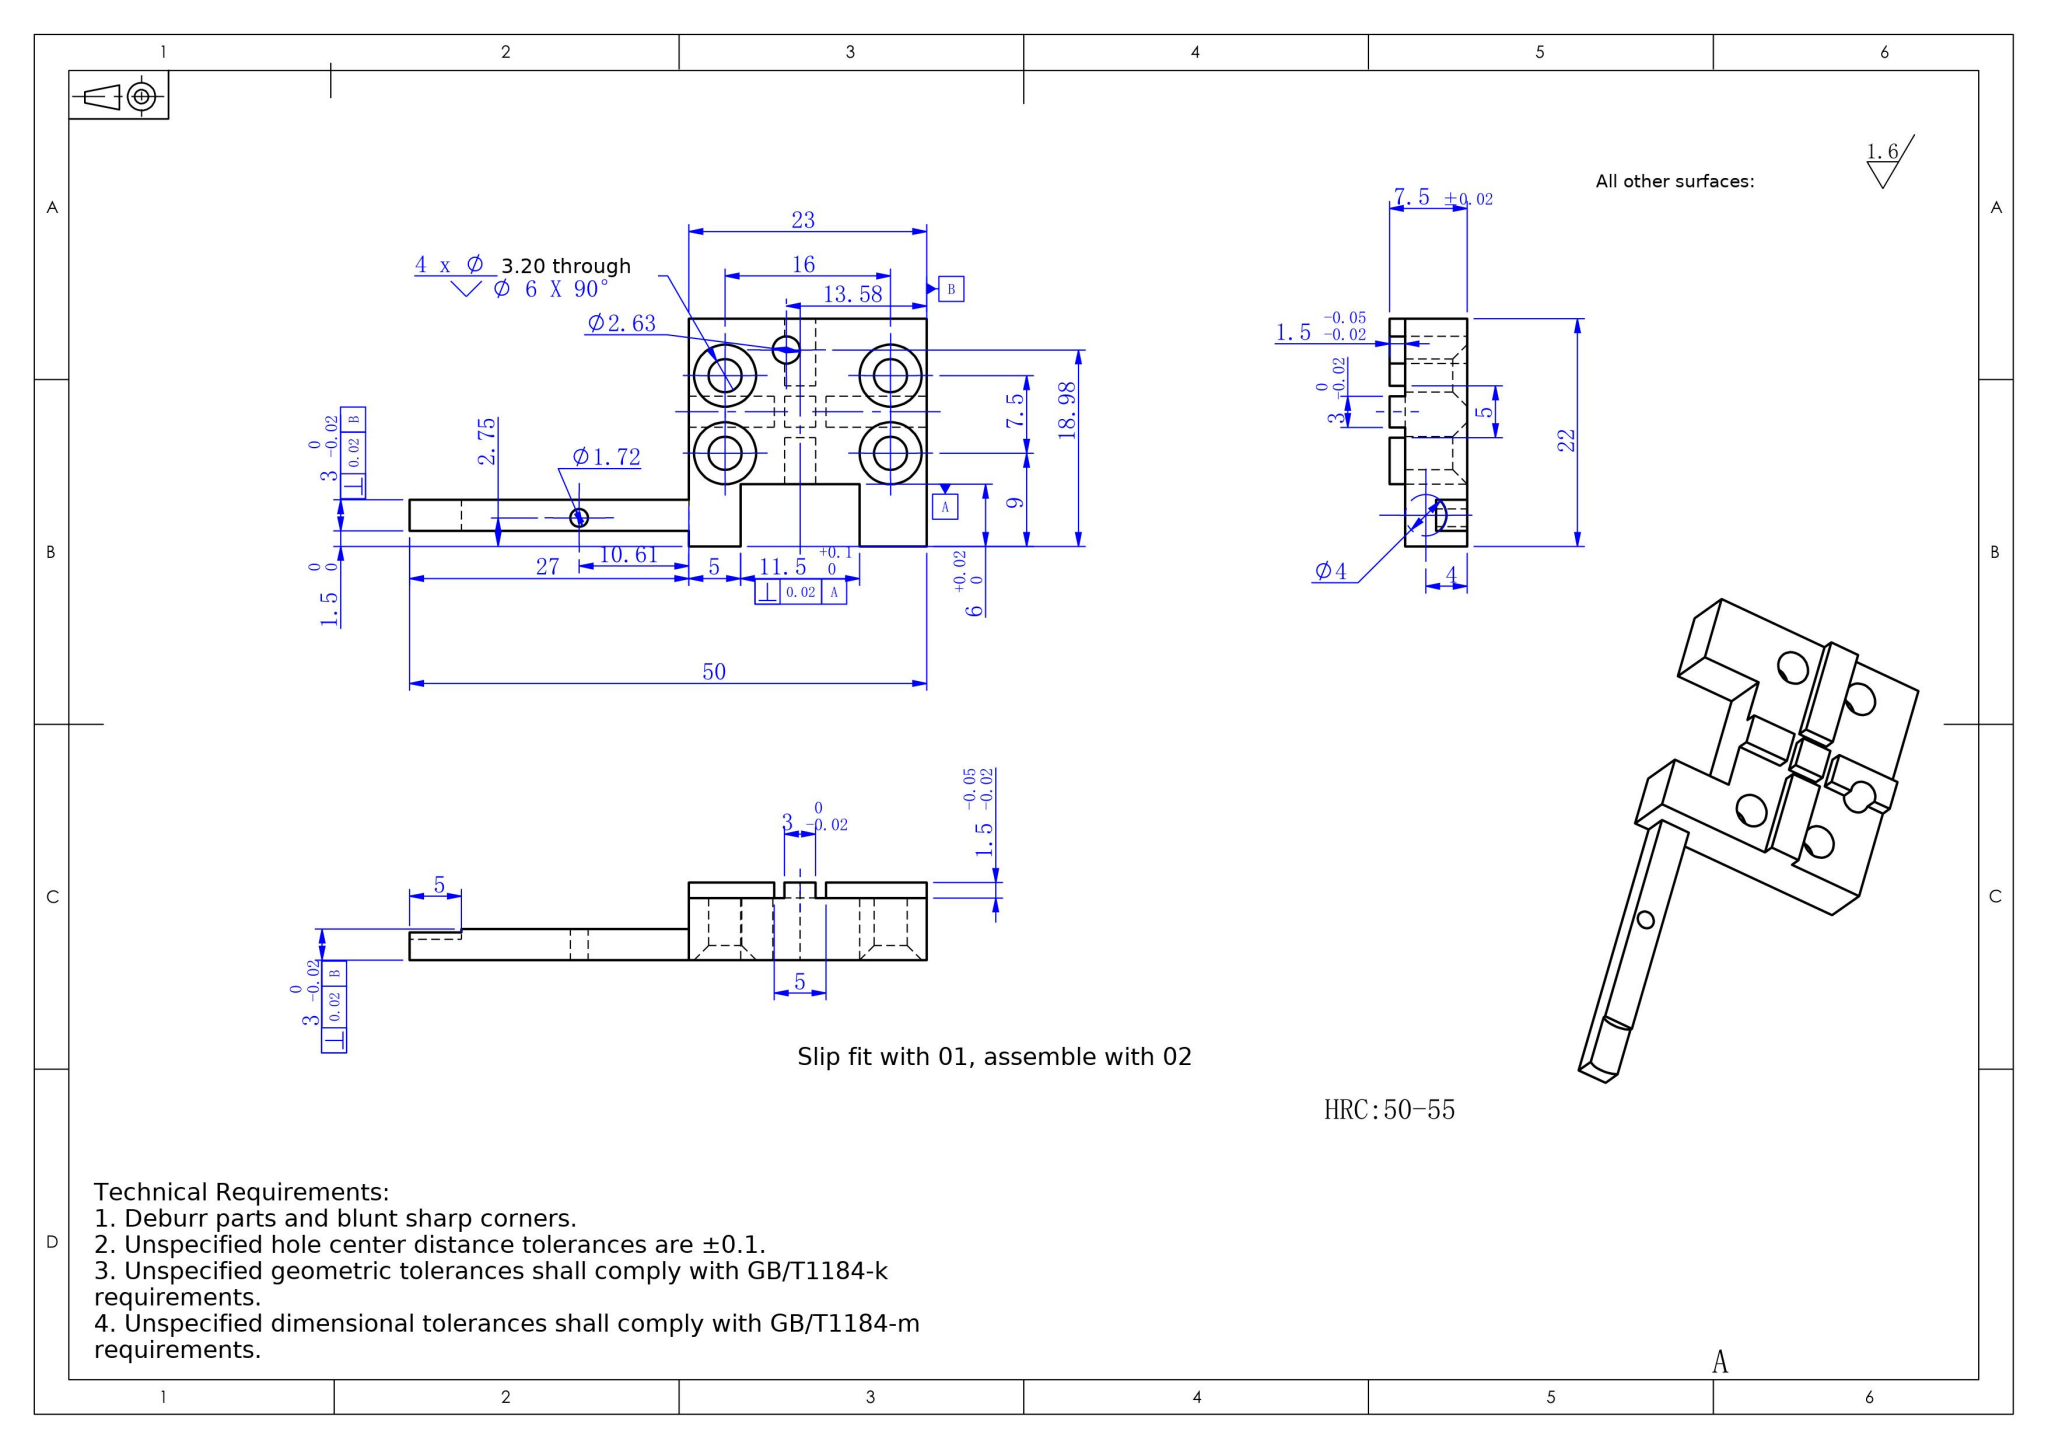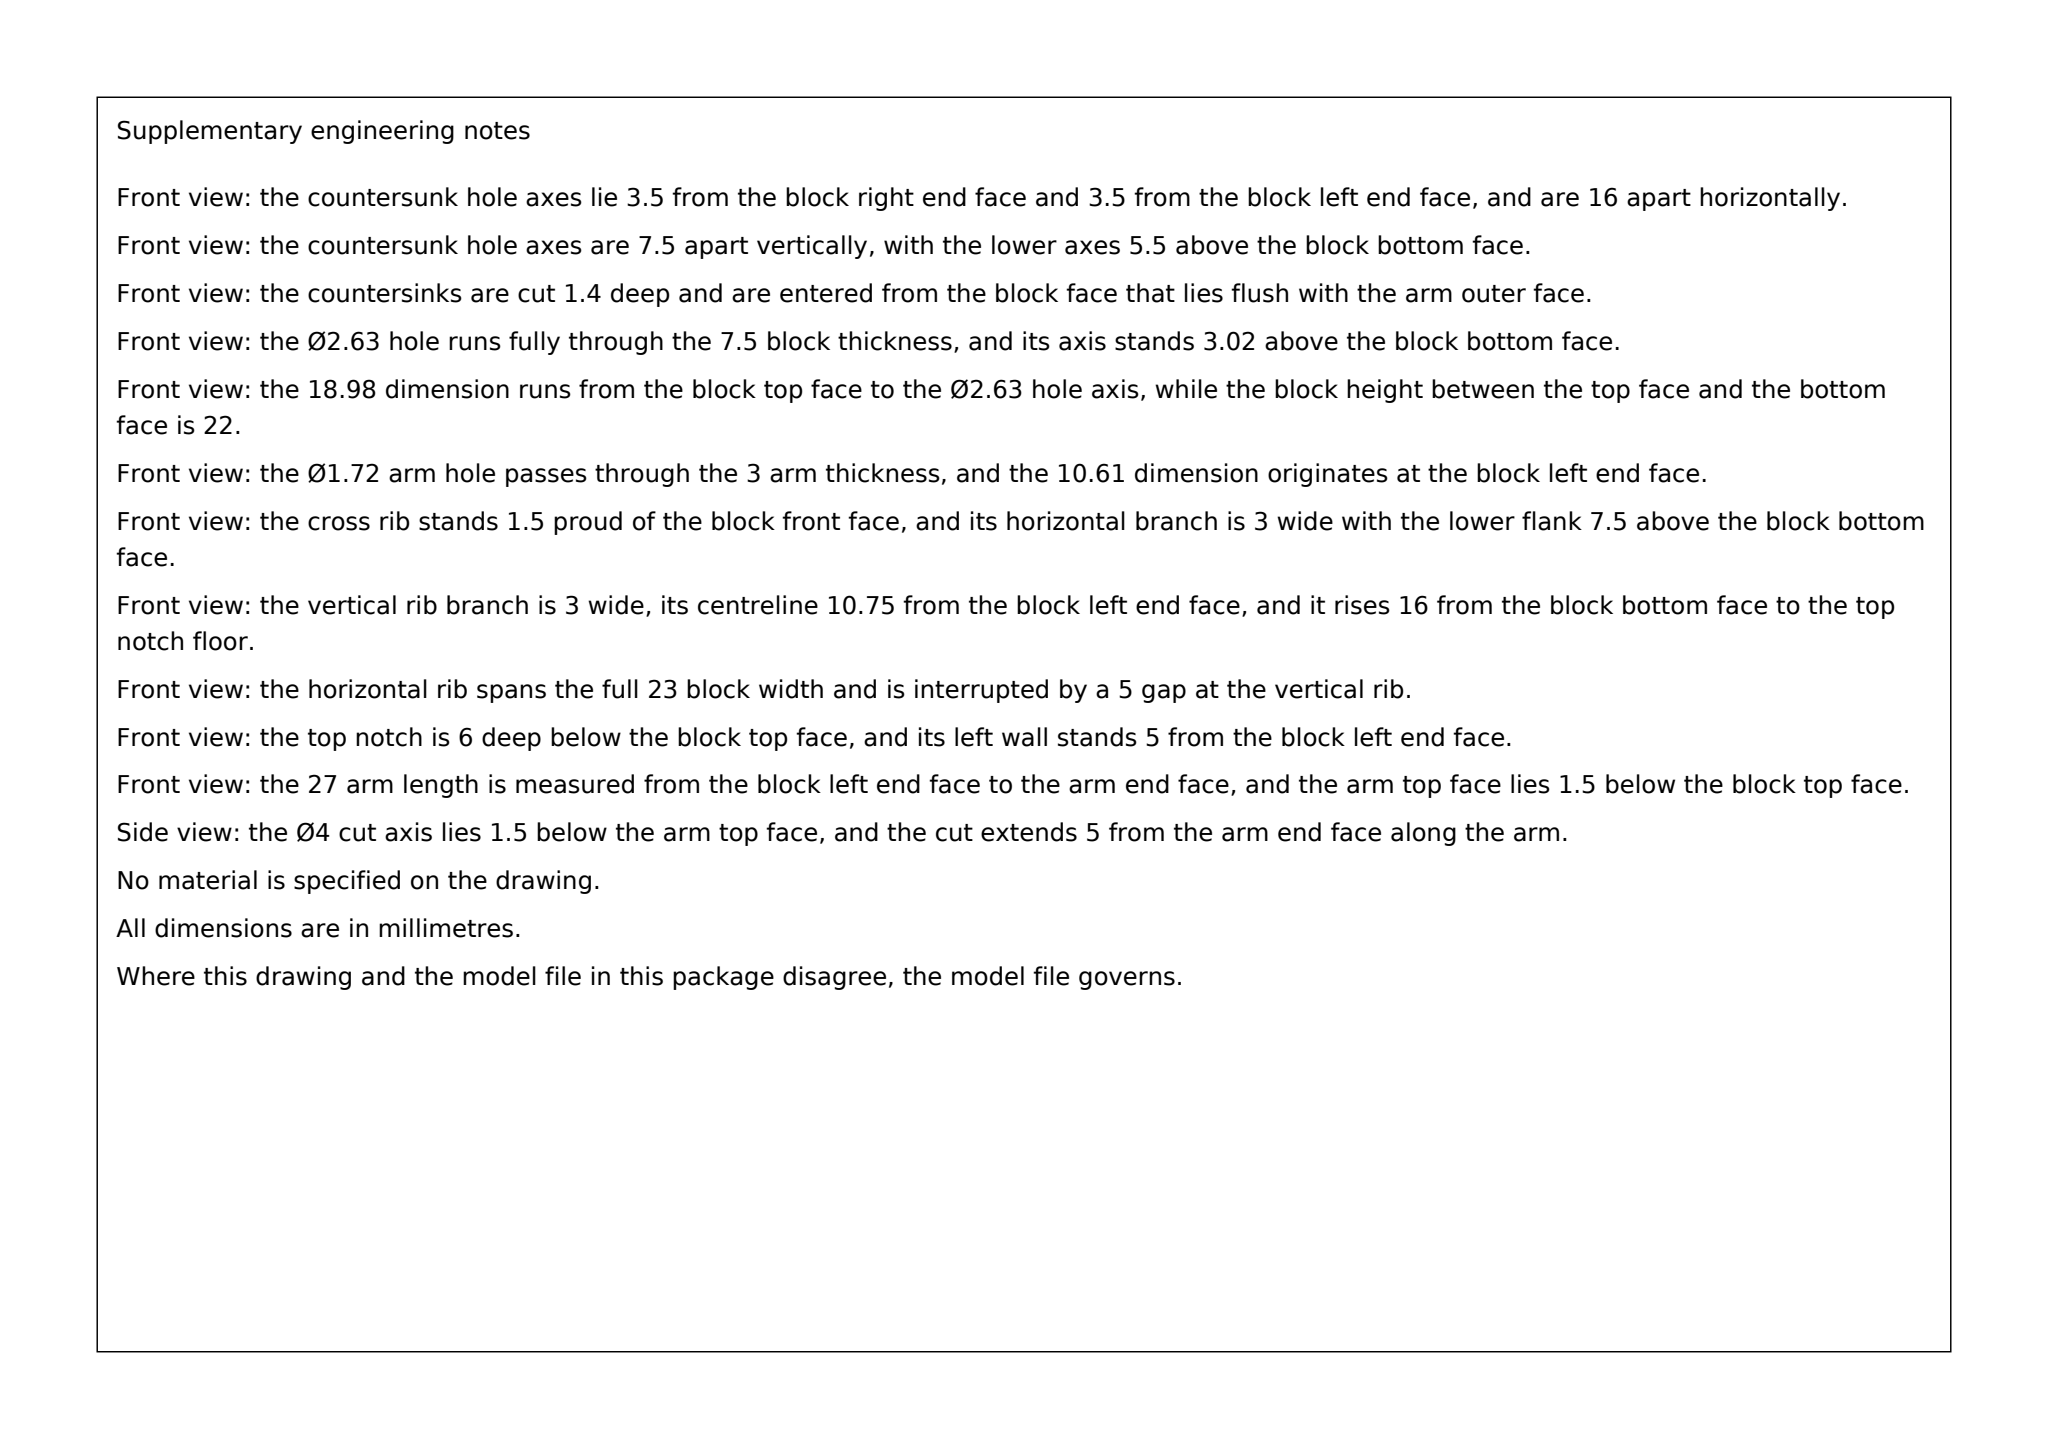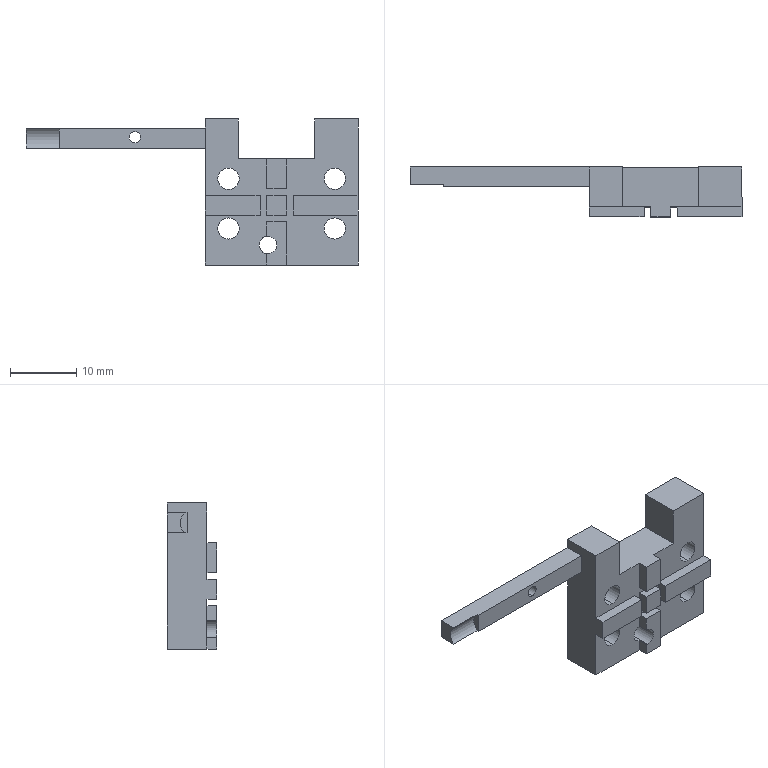Part | SolidWorks | mm | 1 solid | 58 faces | box 50 x 7.5 x 22 mm | volume 2709 mm3 | plane 37 | cylinder 13 | cone 8 | commonest cylinder face diameters 3.2 x8 2.631 x2 1.717 x2 4 x1
Drawing notes:
Central cross-slot, 3 wide through part: slot faces located 36.25 and 39.25 from the left end face of the arm (x=0). | from the solid: axis_planes x=36.25 (4 faces) and x=39.25 (3 faces), 3 mm apart
Bottom-centre notch: floor plane 6.5 above the bottom face (z=0), i.e. notch depth 6.5 from z=0. | from the solid: axis_planes z=0.0 and z=6.5
Ø4 cross-hole in arm, axis parallel to X, 5 deep from the arm end face (x=0); axis 3.5 from datum face y=0 and 19.0 above bottom face z=0. | from the solid: cylinders [4.0,'x',[null,3.5,19.0],5.0]
Ø1.72 pin hole in arm: axis parallel to Y, 16.39 from left end face x=0 and 19.25 above bottom face z=0; depth 3. | from the solid: cylinders [1.717,'y',[16.39,null,19.25],3.0]
Ø2.63 hole: axis parallel to Y, 36.42 from left end face x=0 and 3.02 above bottom face z=0, through 7.5 width. | from the solid: cylinders [2.631,'y',[36.42,null,3.02],7.5]
HORIZONTAL BRANCH OF CENTRAL CROSS-SLOT: 3 HIGH, FLOOR 7.5 AND ROOF 10.5 ABOVE BOTTOM FACE Z=0. | from the solid: axis_planes z=7.5 (x3) and z=10.5 (x3)
3 WIDE THROUGH CROSS-SLOT (X=36.25 TO 39.25 FROM DATUM A): VERTICAL BRANCH RUNS FROM Z=11.5 TO Z=16 ABOVE BOTTOM FACE Z=0, 4.5 HIGH. | from the solid: axis_planes z=11.5 and z=16.0 with x=36.25 / x=39.25
WIDENED SLOT POCKET: 5 LONG, FROM 35.25 TO 40.25 FROM LEFT END FACE (DATUM A, X=0). | from the solid: axis_planes x=35.25 and x=40.25
4X Ø3.20 THRU, CSK Ø6 X 90°: HOLE AXES AT X=30.5 AND X=46.5 FROM DATUM A (LEFT END FACE X=0), 16 APART; NEAREST AXIS 3.5 FROM RIGHT END FACE X=50. | from the solid: cylinders dia 3.2 axis y at x=30.5 and 46.5; bbox_xyz x=50
4X Ø3.20 CSK HOLE AXES AT Z=5.5 AND Z=13.0 ABOVE BOTTOM FACE Z=0 (7.5 APART); COUNTERSINKS ON FACE Y=7.5. | from the solid: cylinders dia 3.2 at z=13.0 and z=5.5; cones 90° ref dia 6 at y=6.1
ARM BAR SECTION IS 3 HIGH: FACES AT Z=17.5 AND Z=20.5 ABOVE BOTTOM FACE Z=0 (DATUM), OVER X=0 TO 27 FROM DATUM A. | from the solid: axis_planes z=17.5 and z=20.5, extent x[0,27] y[4.5,7.5]
ARM BAR IS 3 THICK IN Y: INNER FACE 4.5 FROM DATUM B FACE Y=0; OUTER FACE FLUSH WITH THE Y=7.5 SIDE FACE. | from the solid: axis_plane y=4.5, extent x[5,27] z[17.5,20.5]; axis_plane y=7.5 extent x[0,50] z[0,22]
ARM END RELIEF X=0 TO 5: Ø4 PARTIAL BORE (97° ARC) CUT INTO ARM SIDE, AXIS PARALLEL TO X AT Y=3.5 FROM DATUM B AND Z=19.0 ABOVE BOTTOM FACE Z=0; REMAINING ARM END FACE AT X=0 IS Y=4.8 TO 7.5 BY Z=17.5 TO 20.5. | from the solid: cylinder concave arc Ø4 axis x at (y=3.5, z=19.0) from x=0 to 5, arc 97°; axis_plane x=0 extent y[4.8,7.5] z[17.5,20.5]; axis_plane x=5 extent y[4.5,5.5] z[17.5,20.5]
TOP SLOT IN BLOCK: 11.5 WIDE BETWEEN X=32 AND X=43.5 FROM DATUM A, FLOOR AT Z=16 ABOVE BOTTOM FACE Z=0, I.E. 6 DEEP FROM TOP FACE Z=22; FULL ACROSS Y=1.5 TO 7.5. | from the solid: axis_planes x=32 and x=43.5 extent y[1.5,7.5] z[16,22]; axis_plane z=16 extent x[32,43.5] y[0,7.5]; bbox height 22
build123d program:
from build123d import *

# Parameters (mm, degrees)
SKETCH1_W                                            = 23
SKETCH1_H                                            = 50
BOSS_EXTRUDE1_DEPTH                                  = 20
SKETCH2_W                                            = 6
SKETCH2_H                                            = 5
CUT_EXTRUDE1_DEPTH                                   = 18
SKETCH3_W                                            = 11.5
SKETCH3_H                                            = 50
CUT_EXTRUDE2_DEPTH                                   = 6
SKETCH4_W                                            = 6
SKETCH4_H                                            = 3
BOSS_EXTRUDE2_DEPTH                                  = 27
SKETCH5_W                                            = 1.5
SKETCH5_H                                            = 3
CUT_EXTRUDE3_DEPTH                                   = 27
SKETCH6_R                                            = 2
CUT_EXTRUDE4_DEPTH                                   = 5
SKETCH7_W                                            = 20
SKETCH7_H                                            = 44
CUT_EXTRUDE5_DEPTH                                   = 50.845
SKETCH8_W                                            = 3
SKETCH8_H                                            = 14
BOSS_EXTRUDE3_DEPTH                                  = 1.5
SKETCH9_W                                            = 23
SKETCH9_H                                            = 3
BOSS_EXTRUDE4_DEPTH                                  = 1.5
SKETCH10_W                                           = 1
SKETCH10_H                                           = 14
CUT_EXTRUDE7_DEPTH                                   = 135.519
SKETCH11_W                                           = 23
SKETCH11_H                                           = 1
CUT_EXTRUDE8_DEPTH                                   = 1.5
M3_PHILLIPS_COUNTERSUNK_HEAD_SCREW_TAPER_D           = 3.2
M3_PHILLIPS_COUNTERSUNK_HEAD_SCREW_TAPER_CSINK_D     = 6
M3_PHILLIPS_COUNTERSUNK_HEAD_SCREW_TAPER_CSINK_ANGLE = 90
BOSS_EXTRUDE5_DEPTH                                  = 2
SKETCH17_R                                           = 1.316
SKETCH17_R_2                                         = 0.8586
CUT_EXTRUDE9_DEPTH                                   = 10


with BuildPart() as part:
    # Sketch1 → Boss-Extrude1 (new body)
    with BuildSketch(Plane.XY):
        with Locations((-94.388, -11.818)):
            Rectangle(SKETCH1_W, SKETCH1_H)
    extrude(amount=BOSS_EXTRUDE1_DEPTH)

    # Sketch2 → Cut-Extrude1 (cut)
    with BuildSketch(Plane(origin=(-82.888, 0, 0), x_dir=(0, 0, -1), z_dir=(1, 0, 0))):
        with Locations((-17, -24.318)):
            Rectangle(SKETCH2_W, SKETCH2_H)
    extrude(amount=-CUT_EXTRUDE1_DEPTH, mode=Mode.SUBTRACT)

    # Sketch3 → Cut-Extrude2 (cut)
    with BuildSketch(Plane.XY.offset(20)):
        with Locations((-95.138, -11.818)):
            Rectangle(SKETCH3_W, SKETCH3_H)
    extrude(amount=-CUT_EXTRUDE2_DEPTH, mode=Mode.SUBTRACT)

    # Sketch4 → Boss-Extrude2 (add)
    with BuildSketch(Plane.ZY.offset(105.888)):
        with Locations((17, 11.682)):
            Rectangle(SKETCH4_W, SKETCH4_H)
    extrude(amount=BOSS_EXTRUDE2_DEPTH)

    # Sketch5 → Cut-Extrude3 (cut)
    with BuildSketch(Plane.ZY.offset(132.888)):
        with Locations((19.25, 11.682)):
            Rectangle(SKETCH5_W, SKETCH5_H)
        with Locations((14.75, 11.682)):
            Rectangle(SKETCH5_W, SKETCH5_H)
    extrude(amount=-CUT_EXTRUDE3_DEPTH, mode=Mode.SUBTRACT)

    # Sketch6 → Cut-Extrude4 (cut)
    with BuildSketch(Plane.ZY.offset(132.888)):
        with Locations((17, 9.182)):
            Circle(SKETCH6_R)
    extrude(amount=-CUT_EXTRUDE4_DEPTH, mode=Mode.SUBTRACT)

    # Sketch7 → Cut-Extrude5 (cut, through all)
    with BuildSketch(Plane.ZY.offset(105.888)):
        with Locations((10, -14.818)):
            Rectangle(SKETCH7_W, SKETCH7_H)
    extrude(amount=-CUT_EXTRUDE5_DEPTH, mode=Mode.SUBTRACT)

    # Sketch8 → Boss-Extrude3 (add)
    with BuildSketch(Plane(origin=(0, 7.182, 0), x_dir=(-1, 0, 0), z_dir=(0, -1, 0))):
        with Locations((95.138, -7)):
            Rectangle(SKETCH8_W, SKETCH8_H)
    extrude(amount=BOSS_EXTRUDE3_DEPTH)

    # Sketch9 → Boss-Extrude4 (add)
    with BuildSketch(Plane(origin=(0, 7.182, 0), x_dir=(-1, 0, 0), z_dir=(0, -1, 0))):
        with Locations((94.388, -7)):
            Rectangle(SKETCH9_W, SKETCH9_H)
    extrude(amount=BOSS_EXTRUDE4_DEPTH)

    # Sketch10 → Cut-Extrude7 (cut, through all)
    with BuildSketch(Plane(origin=(0, 7.182, 0), x_dir=(-1, 0, 0), z_dir=(0, -1, 0))):
        with Locations((97.138, -7)):
            Rectangle(SKETCH10_W, SKETCH10_H)
        with Locations((93.138, -7)):
            Rectangle(SKETCH10_W, SKETCH10_H)
    extrude(amount=CUT_EXTRUDE7_DEPTH, mode=Mode.SUBTRACT)

    # Sketch11 → Cut-Extrude8 (cut)
    with BuildSketch(Plane(origin=(0, 5.682, 0), x_dir=(-1, 0, 0), z_dir=(0, -1, 0))):
        with Locations((94.388, -9)):
            Rectangle(SKETCH11_W, SKETCH11_H)
        with Locations((94.388, -5)):
            Rectangle(SKETCH11_W, SKETCH11_H)
    extrude(amount=-CUT_EXTRUDE8_DEPTH, mode=Mode.SUBTRACT)

    # M3 Phillips Countersunk Head Screw Taper (through all)
    with Locations(Plane(origin=(0, 13.182, 0), x_dir=(1, 0, 0), z_dir=(0, 1, 0))):
        with Locations((-86.388, -11), (-102.388, -11), (-86.388, -3.5), (-102.388, -3.5)):
            CounterSinkHole(M3_PHILLIPS_COUNTERSUNK_HEAD_SCREW_TAPER_D / 2, M3_PHILLIPS_COUNTERSUNK_HEAD_SCREW_TAPER_CSINK_D / 2, counter_sink_angle=M3_PHILLIPS_COUNTERSUNK_HEAD_SCREW_TAPER_CSINK_ANGLE)

    # Sketch15 → Boss-Extrude5 (add)
    with BuildSketch(Plane(origin=(0, 0, 0), x_dir=(-1, 0, 0), z_dir=(0, 0, -1))):
        Polygon((82.888, 13.182), (82.888, 7.182), (93.638, 7.182), (93.638, 5.682), (96.638, 5.682), (96.638, 7.182), (105.888, 7.182), (105.888, 13.182), align=None)
    extrude(amount=BOSS_EXTRUDE5_DEPTH)

    # Sketch17 → Cut-Extrude9 (cut)
    with BuildSketch(Plane(origin=(0, 13.182, 0), x_dir=(1, 0, 0), z_dir=(0, 1, 0))):
        with Locations(Location((-96.464, -1.022, 0), (0, 0, 270))):
            Circle(SKETCH17_R)
        with Locations(Location((-116.499, -17.249, 0), (0, 0, 270))):
            Circle(SKETCH17_R_2)
    extrude(amount=-CUT_EXTRUDE9_DEPTH, mode=Mode.SUBTRACT)


solid = part.part